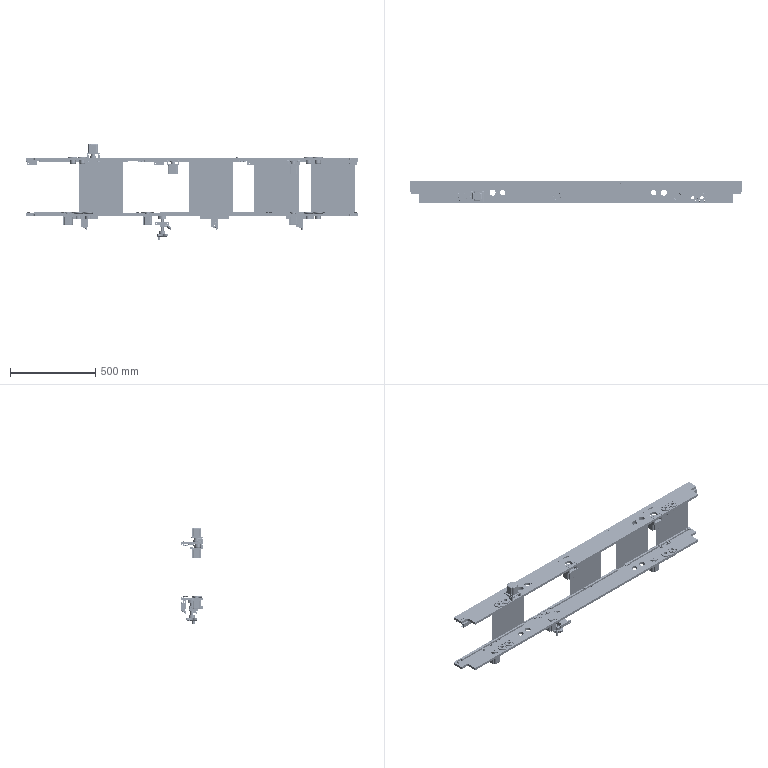Assembly | SolidWorks | mm | 127 component files | 127 solids | 6871 faces | box 1950 x 128 x 564.8 mm | volume 9759573 mm3 | cylinder 2934 | plane 2677 | torus 620 | cone 572 | spline 56 | sphere 12 | commonest cylinder face diameters 5 x216 7 x210 14 x194 63 x180 5.5 x170 4 x161 3.3 x158 10 x138
Bill of materials:
SL010-02047843SupportBar1-1 | 1 | White POM | Long, slender straight bar with a rectangular cross-section. It has three round holes through its wider face: one near each end and one at the middle.
SL010-02047843SupportBar1-1 | 3 | White POM | Long, slender straight bar of rectangular section with three through holes along its length: one near each end and one at the middle.
SL010-02047844SupportBar2-1 | 2 | White POM | Long, slender straight bar of rectangular section with three through holes, one near each end and one at the center. It looks essentially the same as unnamed part.
SL010-02047858StopBarNo.3-1 | 2 | White POM | Long rectangular bar with angled chamfers at both ends of one long edge. The middle section is reduced in height, giving a stepped recess. Four small elongated holes or slots pass through the wide side face.
SL010-02047858StopBarNo.4-1 | 1 | White POM | Long rectangular bar with angled end chamfers, four small elongated holes through the wide face, and a reduced-height recessed section offset toward one end.
SL010-B602-1 | 1 | 45 | Thick annular ring with a central through bore and a concentric annular groove cut into one flat face. The opposite face is flat.
SL010-_CLDM5_25_B_1_2-1 | 1 |  | Stepped cylindrical pin: a long small-diameter shank, a larger cylindrical collar, and a medium-diameter section ending in a hexagonal socket recess. The ends are chamfered or rounded.
SL010-_CLDM5_8_B_2_4-1 | 1 |  | Lever or crank arm: a cylindrical hub with a through bore, joined to a flat, tapered, curved arm that ends in a rounded tip.
SL010-HBA41-D63-1 | 1 |  | Wheel or knob with a finely toothed or knurled rim, a raised split-clamp hub with a central bore, and an off-center cylindrical pin on the underside.
SL010-LXFB-0102009-1 | 1 | Aluminum-6061 | Flanged ring or collar with a stepped (counterbored) central bore and four through holes equally spaced on a bolt circle. The outer edges are chamfered.
SL010-LXFB-0102010-1 | 1 | S45C | Rectangular plate block with a stepped, flanged (T-shaped) profile. The upper body has a large counterbored hole and two small holes. The wider base flange has horizontal through holes at its ends. The top corners are chamfered.
SL010-LXFB-0102011-1 | 1 | Aluminum-6061 | Rectangular block shaft clamp with a large through bore. A slit runs from the bore to one end, and a slot extends partway toward the other end. The block also has two through holes and a cross hole through the side, perpendicular to the slit.
SL010-LXFB-0102017-1 | 1 | S45C | Stepped cylindrical shaft: a long main section with reduced-diameter journals at both ends. One end has a circumferential groove near the tip.
SL010-C-LHFR20-2-1 | 8 |  | Flanged cylindrical bushing: a round flange with four through holes evenly spaced around a central through bore, and a plain cylindrical shank below it.
SL010-LXFB-010203-002-1 | 1 | Aluminum-6061 | Long, thin, flat plate with stepped or notched ends and a row of features along its length: several larger circular holes, many small holes and a few short slots.
SL010-LeadshineStepper-2-1 | 6 |  | Box-like body with a square front flange (chamfered corners) and a through hole at each corner, a raised circular boss in the middle, and a single cylindrical shaft sticking out of the boss.
SL010-LXFB-020200-007-1 | 3 | S45C | Pulley-like rotational part: a cylindrical body between two thin raised rims, a smaller cylindrical hub on one side with two radial holes in a line, and a small central through bore.
SL010-FL625ZZ-1 | 48 |  | Stepped annular part: a thin, wider base flange under a taller cylindrical ring with rounded top edge, a central through bore with a raised inner ring, and a shallow annular groove near the outer top edge.
SL010-LXFB-020200-020-1 | 3 | Aluminum-6061 | Flat T-shaped plate: a wide top bar with angled upper corners, and a narrower central stem with two holes in a line; inner corners are filleted. Edge views show a step in thickness or a joggle between the bar and the stem.
SL010-Material | 4 |  | Thin, plain rectangular sheet with no visible holes or features.
SL010-0ALk-010000-006-2-1 | 3 | 45 | Pulley-like rotational part: a cylindrical band between two thin rims, a smaller coaxial hub with two radial holes in a line, a chamfered hub end, and a small central through bore.
SL010-LXFB-0102007-1 | 3 | Aluminum-6061 | Square flat plate with small corner chamfers, a large central circular opening, four smaller through holes and four larger through holes.
SL010-LXFB-0102008-1 | 6 | Aluminum-6061 | Rectangular block with chamfered edges and two parallel through holes in its top face.
SL010-GB6171-86 M4-1 | 1 |  | Hexagonal nut-like part: chamfered on both faces, with a central round through bore.
SL010-LXFB-010202-003-1 | 2 | S45C | Long, slender bar with a rectangular cross-section, three small elongated holes through the narrow face (one at each end and one at mid-length), and angled cuts at the ends.
SL010-LXFB-010202-01 | 1 | S45C | Long, slender solid bar with a rectangular cross-section. It has three small slotted holes through one face, one near each end and one at mid-length. The bottom corners at both ends are chamfered or beveled.
SL010-LXFB-010203-01 | 1 | Aluminum-6061 | Long, thin flat plate with a rectangular notch or step at each end. Along the plate are three groups of round holes of different sizes, short slots, and many small holes. The pattern looks symmetric about the middle.
SL010-0ALk-010000-012-2-1 | 4 | 304 | Bracket bent from a uniform-thickness sheet into a C or U shape: a long top flange, a vertical web, and a shorter bottom flange. The top flange has a long slot with rounded ends. The web has a square cutout. The bottom flange has a single round hole, which may be countersunk or counterbored.
SL010-E3Z_D61-1 | 4 |  | Rectangular block body with a cylindrical stub on one end. A long, thin rod or cable extends from the body at an angle. There are two round through holes on the top face, and small cylindrical bosses and a rounded tab on one side face. The body outline has one chamfered corner.
Mates:
1. coincident | SL010-RightStreamline-1-1/SL010-LXFB-010203-01-1 face at (-975, -109.904, -316.035) dir (0, 1, 0) | SL010-LeftStreamline-1-1/SL010-LXFB-010203-002-1-1 face at (975, -109.904, -658.035) dir (0, 1, 0)
2. coincident | SL010-RightStreamline-1-1/SL010-LXFB-010203-01-1 face at (-975, -109.904, -316.035) dir (-1, 0, 0) | SL010-LeftStreamline-1-1/SL010-LXFB-010203-002-1-1 face at (-975, -109.904, -658.035) dir (-1, 0, 0)
3. distance | SL010-LeftStreamline-1-1/SL010-LXFB-010203-002-1-1 face at (0, -169.404, -643.035) dir (0, 0, 1) | SL010-RightStreamline-1-1/SL010-LXFB-010203-01-1 face at (0, -169.404, -331.035) dir (0, 0, -1)
4. coincident | SL010-Material-2 face at (110, -107.904, -487.035) dir (0, 1, 0) | SL010-Material-1 face at (-535, -107.904, -487.035) dir (0, 1, 0)
5. coincident | SL010-Material-2 face at (-12, -108.004, -345.035) dir (0, 0, -1) | SL010-Material-1 face at (-657, -108.004, -345.035) dir (0, 0, -1)
6. distance | SL010-RightStreamline-1-1/SL010-02047843SupportBar1-1-1 face at (898.47, -111.404, -341.035) dir (0, 1, 0) | SL010-Material-4 face at (827.087, -109.904, -487.035) dir (0, -1, 0)
7. width | SL010-Material-4 face at (697.087, -107.904, -637.035) dir (0, 0, -1) | SL010-Material-4 face at (697.087, -107.904, -337.035) dir (0, 0, 1) | SL010-RightStreamline-1-1/SL010-LXFB-010203-01-1 face at (0, -169.404, -316.035) dir (0, 0, 1) | SL010-LeftStreamline-1-1/SL010-LXFB-010203-002-1-1 face at (0, -169.404, -658.035) dir (0, 0, -1)
8. coincident | SL010-Material-4 face at (827.087, -107.904, -487.035) dir (0, 1, 0) | SL010-Material-2 face at (110, -107.904, -487.035) dir (0, 1, 0)
9. coincident | SL010-Material-4 edge at (705.087, -107.904, -345.035) dir (1, 0, 0) | SL010-Material-2 face at (-12, -108.004, -345.035) dir (0, 0, -1)
10. coincident | SL010-Material-4 face at (827.087, -107.904, -487.035) dir (0, 1, 0) | SL010-Material-3 face at (496.654, -107.904, -487.035) dir (0, 1, 0)
11. coincident | SL010-Material-4 face at (705.087, -108.004, -345.035) dir (0, 0, -1) | SL010-Material-3 edge at (374.654, -108.004, -345.035) dir (1, 0, 0)
12. concentric | SL010-LXFB-010203-002-1-1 face at (732.973, 100.193, 1492.5) dir (0, 0, -1) r 2.1 | SL010-PulleyAssembly-1-1/SL010-FL625ZZ-1-2 face at (732.973, 100.193, 1470.5) dir (0, 0, 1) r 2.5
13. distance | SL010-PulleyAssembly-1-1/SL010-FL625ZZ-1-1 face at (732.881, 107.193, 1491.5) dir (0, 0, 1) | SL010-LXFB-010203-002-1-1 face at (-227.027, 50.193, 1492.5) dir (0, 0, -1)
14. concentric | SL010-LXFB-010203-002-1-1 face at (532.973, 84.193, 1492.5) dir (0, 0, -1) r 2.1 | SL010-PulleyAssembly-1-2/SL010-FL625ZZ-1-2 face at (532.973, 84.193, 1470.5) dir (0, 0, 1) r 2.5
15. coincident | SL010-PulleyAssembly-1-1/SL010-FL625ZZ-1-2 face at (733.036, 107.193, 1481.5) dir (0, 0, -1) | SL010-PulleyAssembly-1-2/SL010-FL625ZZ-1-2 face at (533.02, 91.193, 1481.5) dir (0, 0, -1)
16. coincident | SL010-PulleyAssembly-1-1/SL010-FL625ZZ-1-2 face at (733.036, 107.193, 1481.5) dir (0, 0, -1) | SL010-PulleyAssembly-1-3/SL010-FL625ZZ-1-2 face at (473.371, 91.182, 1481.5) dir (0, 0, -1)
17. slot | SL010-PulleyAssembly-1-3/SL010-FL625ZZ-1-2 face at (472.973, 84.193, 1470.5) dir (0, 0, 1) r 2.5 | SL010-LXFB-010203-002-1-1 face at (455.723, 84.193, 1507.5) dir (0, 0, 1) r 2.75
18. coincident | SL010-PulleyAssembly-1-1/SL010-FL625ZZ-1-2 face at (733.036, 107.193, 1481.5) dir (0, 0, -1) | SL010-PulleyAssembly-1-7/SL010-FL625ZZ-1-2 face at (31.14, 94.439, 1481.5) dir (0, 0, -1)
19. slot | SL010-PulleyAssembly-1-13/SL010-FL625ZZ-1-2 face at (3.973, 84.193, 1470.5) dir (0, 0, 1) r 2.5 | SL010-LXFB-010203-002-1-1 face at (-13.277, 81.443, 1507.5) dir (0, 1, 0)
20. concentric | SL010-LXFB-010203-002-1-1 face at (-668.027, 100.193, 1492.5) dir (0, 0, -1) r 2.1 | SL010-PulleyAssembly-1-8/SL010-FL625ZZ-1-2 face at (-668.027, 100.193, 1470.5) dir (0, 0, 1) r 2.5
21. concentric | SL010-LXFB-010203-002-1-1 face at (-687.027, 100.193, 1492.5) dir (0, 0, -1) r 2.1 | SL010-PulleyAssembly-1-9/SL010-FL625ZZ-1-2 face at (-687.027, 100.193, 1470.5) dir (0, 0, 1) r 2.5
22. coincident | SL010-PulleyAssembly-1-1/SL010-FL625ZZ-1-2 face at (733.036, 107.193, 1481.5) dir (0, 0, -1) | SL010-PulleyAssembly-1-8/SL010-FL625ZZ-1-2 face at (-667.964, 107.193, 1481.5) dir (0, 0, -1)
23. coincident | SL010-PulleyAssembly-1-1/SL010-FL625ZZ-1-2 face at (733.036, 107.193, 1481.5) dir (0, 0, -1) | SL010-PulleyAssembly-1-6/SL010-FL625ZZ-1-2 face at (88.551, 106.566, 1481.5) dir (0, 0, -1)
24. concentric | SL010-LXFB-010203-002-1-1 face at (63.973, 84.193, 1492.5) dir (0, 0, -1) r 2.1 | SL010-PulleyAssembly-1-12/SL010-FL625ZZ-1-2 face at (63.973, 84.193, 1470.5) dir (0, 0, 1) r 2.5
25. coincident | SL010-PulleyAssembly-1-1/SL010-FL625ZZ-1-2 face at (733.036, 107.193, 1481.5) dir (0, 0, -1) | SL010-PulleyAssembly-1-12/SL010-FL625ZZ-1-2 face at (64.036, 91.193, 1481.5) dir (0, 0, -1)
26. coincident | SL010-PulleyAssembly-1-1/SL010-FL625ZZ-1-2 face at (733.036, 107.193, 1481.5) dir (0, 0, -1) | SL010-PulleyAssembly-1-13/SL010-FL625ZZ-1-2 face at (4.977, 91.121, 1481.5) dir (0, 0, -1)
27. coincident | SL010-PulleyAssembly-1-1/SL010-FL625ZZ-1-2 face at (733.036, 107.193, 1481.5) dir (0, 0, -1) | SL010-PulleyAssembly-1-9/SL010-FL625ZZ-1-2 face at (-693.737, 98.198, 1481.5) dir (0, 0, -1)
28. concentric | SL010-LXFB-010203-002-1-1 face at (-942.027, 84.193, 1492.5) dir (0, 0, -1) r 2.1 | SL010-PulleyAssembly-1-14/SL010-FL625ZZ-1-2 face at (-942.027, 84.193, 1470.5) dir (0, 0, 1) r 2.5
29. coincident | SL010-PulleyAssembly-1-1/SL010-FL625ZZ-1-2 face at (733.036, 107.193, 1481.5) dir (0, 0, -1) | SL010-PulleyAssembly-1-14/SL010-FL625ZZ-1-2 face at (-943.982, 90.915, 1481.5) dir (0, 0, -1)
30. slot | SL010-PulleyAssembly-1-15/SL010-FL625ZZ-1-1 face at (-1002.027, 84.193, 1502.5) dir (0, 0, -1) r 2.5 | SL010-LXFB-010203-002-1-1 face at (-1019.277, 84.193, 1507.5) dir (0, 0, 1) r 2.75
31. coincident | SL010-PulleyAssembly-1-1/SL010-FL625ZZ-1-2 face at (733.036, 107.193, 1481.5) dir (0, 0, -1) | SL010-PulleyAssembly-1-15/SL010-FL625ZZ-1-2 face at (-1006.227, 89.793, 1481.5) dir (0, 0, -1)
32. concentric | SL010-LXFB-010203-002-1-1 face at (-1187.027, 100.193, 1492.5) dir (0, 0, -1) r 2.1 | SL010-PulleyAssembly-1-18/SL010-FL625ZZ-1-2 face at (-1187.027, 100.193, 1470.5) dir (0, 0, 1) r 2.5
33. coincident | SL010-PulleyAssembly-1-1/SL010-FL625ZZ-1-2 face at (733.036, 107.193, 1481.5) dir (0, 0, -1) | SL010-PulleyAssembly-1-18/SL010-FL625ZZ-1-2 face at (-1186.964, 107.193, 1481.5) dir (0, 0, -1)
34. coincident | SL010-LXFB-010203-002-1-1 face at (-227.027, 50.193, 1492.5) dir (0, 0, -1) | SL010-02047844SupportBar2-1-1 face at (-316.451, 103.193, 1492.5) dir (0, 0, 1)
35. distance | SL010-02047844SupportBar2-1-1 face at (-36.451, 108.193, 1482.5) dir (0, 1, 0) | SL010-LXFB-010203-002-1-1 face at (-1202.027, 109.693, 1507.5) dir (0, 1, 0)
36. symmetric | SL010-PulleyAssembly-1-7/SL010-FL625ZZ-1-1 face at (35.126, 100.193, 1502.5) dir (0, 0, -1) r 8 | SL010-PulleyAssembly-1-8/SL010-FL625ZZ-1-1 face at (-668.027, 100.193, 1502.5) dir (0, 0, -1) r 8 | SL010-02047844SupportBar2-1-1 plane at (-316.451, 103.193, 1487.5) dir (-1, 0, 0)
37. coincident | SL010-02047843SupportBar1-1-1 face at (-937.027, 103.193, 1482.5) dir (0, 0, -1) | SL010-02047844SupportBar2-1-1 face at (-316.451, 103.193, 1482.5) dir (0, 0, -1)
38. coincident | SL010-02047843SupportBar1-1-1 face at (-697.027, 108.193, 1482.5) dir (0, 1, 0) | SL010-02047844SupportBar2-1-1 face at (-36.451, 108.193, 1482.5) dir (0, 1, 0)
39. symmetric | SL010-PulleyAssembly-1-9/SL010-FL625ZZ-1-1 face at (-687.027, 100.193, 1502.5) dir (0, 0, -1) r 8 | SL010-PulleyAssembly-1-18/SL010-FL625ZZ-1-1 face at (-1187.027, 100.193, 1502.5) dir (0, 0, -1) r 8 | SL010-02047843SupportBar1-1-1 plane at (-937.027, 103.193, 1487.5) dir (-1, 0, 0)
40. concentric | SL010-LXFB-010203-002-1-1 face at (-64.755, 67.421, 1507.5) dir (0, 0, 1) r 2.1 | SL010-2M-0112-000-2-1-1/SL010-LXFB-0102009-1-1 face at (-64.755, 67.421, 1522.5) dir (0, 0, 1) r 2.75
41. concentric | SL010-LXFB-010203-002-1-1 face at (-39.299, 67.421, 1507.5) dir (0, 0, 1) r 2.1 | SL010-2M-0112-000-2-1-1/SL010-LXFB-0102009-1-1 face at (-39.299, 67.421, 1522.5) dir (0, 0, 1) r 5
42. coincident | SL010-LXFB-010203-002-1-1 face at (-227.027, 50.193, 1507.5) dir (0, 0, 1) | SL010-2M-0112-000-2-1-1/SL010-LXFB-0102009-1-1 face at (-52.027, 54.693, 1507.5) dir (0, 0, -1)
43. coincident | SL010-LXFB-010203-002-1-1 face at (-227.027, 50.193, 1507.5) dir (0, 0, 1) | SL010-MotorDriveWheel-1-1/SL010-LeadshineStepper-2-1-1 face at (531.173, -0.05689, 1507.5) dir (0, 0, -1)
44. distance | SL010-MotorDriveWheel-1-1/SL010-LeadshineStepper-2-1-1 face at (474.773, 56.343, 1561.5) dir (0, 1, 0) | SL010-LXFB-010203-002-1-1 face at (-1202.027, 109.693, 1507.5) dir (0, 1, 0)
45. coincident | SL010-LXFB-010203-002-1-1 face at (-227.027, 50.193, 1507.5) dir (0, 0, 1) | SL010-MotorDriveWheel-1-2/SL010-LeadshineStepper-2-1-1 face at (62.173, -0.05689, 1507.5) dir (0, 0, -1)
46. coincident | SL010-MotorDriveWheel-1-1/SL010-LeadshineStepper-2-1-1 face at (474.773, 56.343, 1561.5) dir (0, 1, 0) | SL010-MotorDriveWheel-1-2/SL010-LeadshineStepper-2-1-1 face at (5.773, 56.343, 1561.5) dir (0, 1, 0)
47. coincident | SL010-LXFB-010203-002-1-1 face at (-227.027, 50.193, 1507.5) dir (0, 0, 1) | SL010-MotorDriveWheel-1-3/SL010-LeadshineStepper-2-1-1 face at (-793.827, -0.05689, 1507.5) dir (0, 0, -1)
48. coincident | SL010-LXFB-010203-002-1-1 face at (-227.027, 50.193, 1492.5) dir (0, 0, -1) | SL010-02047843SupportBar1-1-2 face at (442.147, 103.193, 1492.5) dir (0, 0, 1)
49. coincident | SL010-02047844SupportBar2-1-1 face at (-36.451, 108.193, 1482.5) dir (0, 1, 0) | SL010-02047843SupportBar1-1-2 face at (702.147, 108.193, 1482.5) dir (0, 1, 0)
50. coincident | SL010-LXFB-010203-002-1-1 face at (-227.027, 50.193, 1507.5) dir (0, 0, 1) | SL010-02047858StopBarNo.3-1-1 face at (747.973, 109.693, 1507.5) dir (0, 0, 1)
51. coincident | SL010-LXFB-010203-002-1-1 face at (-1202.027, 109.693, 1507.5) dir (0, 1, 0) | SL010-02047858StopBarNo.3-1-1 face at (406.473, 109.693, 1497) dir (0, -1, 0)
52. coincident | SL010-LXFB-010203-002-1-1 face at (747.973, 109.693, 1507.5) dir (1, 0, 0) | SL010-02047858StopBarNo.3-1-1 face at (747.973, 109.693, 1486.5) dir (1, 0, 0)
53. coincident | SL010-LXFB-010203-002-1-1 face at (-227.027, 50.193, 1507.5) dir (0, 0, 1) | SL010-02047858StopBarNo.3-1-2 face at (-519.027, 109.693, 1507.5) dir (0, 0, 1)
54. coincident | SL010-LXFB-010203-002-1-1 face at (-1202.027, 109.693, 1507.5) dir (0, 1, 0) | SL010-02047858StopBarNo.3-1-2 face at (-860.527, 109.693, 1497) dir (0, -1, 0)
55. coincident | SL010-LXFB-010203-002-1-1 face at (-1202.027, 109.693, 1507.5) dir (-1, 0, 0) | SL010-02047858StopBarNo.3-1-2 face at (-1202.027, 109.693, 1486.5) dir (-1, 0, 0)
56. coincident | SL010-02047858StopBarNo.3-1-1 face at (406.473, 117.693, 1497) dir (0, 1, 0) | SL010-02047858StopBarNo.4-1-2 face at (-227.027, 117.693, 1497) dir (0, 1, 0)
57. coincident | SL010-02047858StopBarNo.3-1-1 face at (64.973, 109.693, 1486.5) dir (-1, 0, 0) | SL010-02047858StopBarNo.4-1-2 face at (64.973, 117.693, 1486.5) dir (1, 0, 0)
58. coincident | SL010-LXFB-010203-002-1-1 face at (-227.027, 50.193, 1507.5) dir (0, 0, 1) | SL010-02047858StopBarNo.4-1-2 face at (-519.027, 117.693, 1507.5) dir (0, 0, 1)
59. coincident | SL010-LXFB-010203-002-1-1 face at (-227.027, 50.193, 1507.5) dir (0, 0, 1) | SL010-SideClampAssembly-DB-1-1/SL010-HLQ8X10SAF(0)+(DS1-H-2)-DB-1-1/SL010-HLQ8X10-S-AF-0-rod-DB-1-1 face at (414.973, 103.693, 1507.5) dir (0, 0, -1)
60. distance | SL010-SideClampAssembly-DB-1-1/SL010-LXFB-020200-020-1-1 face at (406.473, 110.193, 1531.5) dir (0, -1, 0) | SL010-LXFB-010203-002-1-1 face at (-1202.027, 109.693, 1507.5) dir (0, 1, 0)
61. width | SL010-SideClampAssembly-DB-1-1/SL010-LXFB-020200-020-1-1 face at (322.723, 116.193, 1570.5) dir (-1, 0, 0) | SL010-SideClampAssembly-DB-1-1/SL010-LXFB-020200-020-1-1 face at (490.223, 116.193, 1570.5) dir (1, 0, 0) | SL010-02047858StopBarNo.3-1-1 face at (321.723, 109.693, 1507.5) dir (1, 0, 0) | SL010-02047858StopBarNo.3-1-1 face at (491.223, 109.693, 1507.5) dir (-1, 0, 0)
62. coincident | SL010-SideClampAssembly-DB-1-1/SL010-LXFB-020200-020-1-1 face at (406.473, 116.193, 1531.5) dir (0, 1, 0) | SL010-SideClampAssembly-DB-1-2/SL010-LXFB-020200-020-1-1 face at (-358.277, 116.193, 1531.5) dir (0, 1, 0)
63. coincident | SL010-LXFB-010203-002-1-1 face at (-227.027, 50.193, 1507.5) dir (0, 0, 1) | SL010-SideClampAssembly-DB-1-2/SL010-HLQ8X10SAF(0)+(DS1-H-2)-DB-1-1/SL010-HLQ8X10-S-AF-0-rod-DB-1-1 face at (-349.777, 103.693, 1507.5) dir (0, 0, -1)
64. width | SL010-SideClampAssembly-DB-1-2/SL010-LXFB-020200-020-1-1 face at (-442.027, 116.193, 1570.5) dir (-1, 0, 0) | SL010-SideClampAssembly-DB-1-2/SL010-LXFB-020200-020-1-1 face at (-274.527, 116.193, 1570.5) dir (1, 0, 0) | SL010-02047858StopBarNo.4-1-2 face at (-273.527, 110.554, 1486.5) dir (-1, 0, 0) | SL010-02047858StopBarNo.4-1-2 face at (-443.027, 110.554, 1486.5) dir (1, 0, 0)
65. coincident | SL010-SideClampAssembly-DB-1-2/SL010-LXFB-020200-020-1-1 face at (-358.277, 116.193, 1531.5) dir (0, 1, 0) | SL010-SideClampAssembly-DB-1-3/SL010-LXFB-020200-020-1-1 face at (-860.527, 116.193, 1531.5) dir (0, 1, 0)
66. coincident | SL010-LXFB-010203-002-1-1 face at (-227.027, 50.193, 1507.5) dir (0, 0, 1) | SL010-SideClampAssembly-DB-1-3/SL010-HLQ8X10SAF(0)+(DS1-H-2)-DB-1-1/SL010-HLQ8X10-S-AF-0-rod-DB-1-1 face at (-852.027, 103.693, 1507.5) dir (0, 0, -1)
67. width | SL010-SideClampAssembly-DB-1-3/SL010-LXFB-020200-020-1-1 face at (-944.277, 116.193, 1570.5) dir (-1, 0, 0) | SL010-SideClampAssembly-DB-1-3/SL010-LXFB-020200-020-1-1 face at (-776.777, 116.193, 1570.5) dir (1, 0, 0) | SL010-02047858StopBarNo.3-1-2 face at (-945.277, 109.693, 1507.5) dir (1, 0, 0) | SL010-02047858StopBarNo.3-1-2 face at (-775.777, 109.693, 1507.5) dir (-1, 0, 0)
68. concentric | SL010-LXFB-010203-002-1-1 face at (-912.027, 19.693, 1492.5) dir (0, 0, 1) r 16 | SL010-C-LHFR20-2-1-1 face at (-912.027, 19.693, 1526.5) dir (0, 0, -1) r 16
69. concentric | SL010-LXFB-010203-002-1-1 face at (-896.825, 34.896, 1507.5) dir (0, 0, 1) r 2.1 | SL010-C-LHFR20-2-1-1 face at (-896.825, 34.896, 1484.5) dir (0, 0, -1) r 4.5
70. coincident | SL010-LXFB-010203-002-1-1 face at (-227.027, 50.193, 1492.5) dir (0, 0, -1) | SL010-C-LHFR20-2-1-1 edge at (-912.027, 19.693, 1492.5) dir (0, 0, -1) r 26.5
71. concentric | SL010-LXFB-010203-002-1-1 face at (-967.027, 19.693, 1492.5) dir (0, 0, 1) r 16 | SL010-C-LHFR20-2-1-2 face at (-967.027, 19.693, 1526.5) dir (0, 0, -1) r 16
72. concentric | SL010-LXFB-010203-002-1-1 face at (-951.825, 34.896, 1507.5) dir (0, 0, 1) r 2.1 | SL010-C-LHFR20-2-1-2 face at (-951.825, 34.896, 1484.5) dir (0, 0, -1) r 4.5
73. coincident | SL010-LXFB-010203-002-1-1 face at (-227.027, 50.193, 1492.5) dir (0, 0, -1) | SL010-C-LHFR20-2-1-2 face at (-955.89, 30.83, 1492.5) dir (0, 0, 1)
74. coincident | SL010-LXFB-010203-002-1-1 face at (-227.027, 50.193, 1492.5) dir (0, 0, -1) | SL010-C-LHFR20-2-1-4 face at (334.11, 30.83, 1492.5) dir (0, 0, 1)
75. coincident | SL010-LXFB-010203-002-1-1 face at (-227.027, 50.193, 1492.5) dir (0, 0, -1) | SL010-C-LHFR20-2-1-3 face at (279.11, 30.83, 1492.5) dir (0, 0, 1)
76. concentric | SL010-LXFB-010203-002-1-1 sketch segment at (3.973, 84.193, 1492.5) dir (0, 0, -1) r 9.639 | SL010-PulleyAssembly-1-13/SL010-FL625ZZ-1-2 face at (3.973, 84.193, 1470.5) dir (0, 0, 1) r 2.5
77. concentric | SL010-LXFB-010203-002-1-1 sketch segment at (-1002.027, 84.193, 1492.5) dir (0, 0, -1) r 11.985 | SL010-PulleyAssembly-1-15/SL010-FL625ZZ-1-2 face at (-1002.027, 84.193, 1470.5) dir (0, 0, 1) r 2.5
78. concentric | SL010-LXFB-010203-002-1-1 sketch segment at (472.973, 84.193, 1492.5) dir (0, 0, -1) r 10.481 | SL010-PulleyAssembly-1-3/SL010-FL625ZZ-1-2 face at (472.973, 84.193, 1470.5) dir (0, 0, 1) r 2.5
79. symmetric | SL010-PulleyAssembly-1-12/SL010-FL625ZZ-1-1 face at (63.973, 84.193, 1502.5) dir (0, 0, -1) r 8 | SL010-PulleyAssembly-1-13/SL010-FL625ZZ-1-1 face at (3.973, 84.193, 1502.5) dir (0, 0, -1) r 8 | SL010-MotorDriveWheel-1-2/SL010-LeadshineStepper-2-1-1 plane at (33.973, 28.143, 1507.5) dir (-1, 0, 0)
80. symmetric | SL010-PulleyAssembly-1-2/SL010-FL625ZZ-1-1 face at (532.973, 84.193, 1502.5) dir (0, 0, -1) r 8 | SL010-PulleyAssembly-1-3/SL010-FL625ZZ-1-1 face at (472.973, 84.193, 1502.5) dir (0, 0, -1) r 8 | SL010-MotorDriveWheel-1-1/SL010-LeadshineStepper-2-1-1 plane at (502.973, 28.143, 1507.5) dir (-1, 0, 0)
81. concentric | SL010-LXFB-010203-002-1-1 face at (-822.027, 28.143, 1507.5) dir (0, 0, -1) r 22.5 | SL010-MotorDriveWheel-1-3/SL010-LXFB-020200-007-1-1 face at (-822.027, 28.143, 1491.9) dir (0, 0, 1) r 18.5
82. coincident | SL010-LXFB-0102009-1-1 face at (0, 25, 37) dir (0, 0, 1) | SL010-B602-1-1 face at (0, 38.7, 37) dir (0, 0, -1)
83. concentric | SL010-LXFB-0102009-1-1 face at (0, 25, 37) dir (0, 0, 1) r 14 | SL010-B602-1-1 face at (0, 25, 45) dir (0, 0, -1) r 6
84. concentric | SL010-B602-1-1 face at (0, 25, 45) dir (0, 0, -1) r 6 | SL010-LXFB-0102017-1-2 face at (0, 25, 37) dir (0, 0, 1) r 6
85. coincident | SL010-B602-1-1 face at (0, 33.8, 37) dir (0, 0, -1) | SL010-LXFB-0102017-1-2 face at (0, 25, 37) dir (0, 0, 1)
86. concentric | SL010-LXFB-0102017-1-2 face at (0, 25, -43) dir (0, 0, 1) r 8 | SL010-LXFB-0102010-1-1 face at (0, 25, 10) dir (0, 0, 1) r 8
87. distance | SL010-LXFB-0102010-1-1 face at (0, 0, -10) dir (0, 0, -1) | SL010-LXFB-0102009-1-1 face at (0, 25, 30) dir (0, 0, -1)
88. coincident | SL010-LXFB-0102010-1-1 face at (0, 0, -10) dir (0, 0, -1) | SL010-LXFB-0102011-1-1 face at (0, 16.5, -10) dir (0, 0, 1)
89. concentric | SL010-LXFB-0102017-1-2 face at (0, 25, -43) dir (0, 0, 1) r 8 | SL010-LXFB-0102011-1-1 face at (0, 25, -20) dir (0, 0, 1) r 8
90. parallel | SL010-LXFB-0102010-1-1 face at (-25, 40, 10) dir (0, 1, 0) | SL010-LXFB-0102011-1-1 face at (-15, 41.5, -10) dir (0, 1, 0)
91. coordinate | SL010-LXFB-0102010-1-1 sketch point at (0, 0, 0) dir (1, 0, 0) | SL010-2M-0112-000-2-1 sketch point at (0, 0, 0) dir (1, 0, 0)
92. angle | SL010-LXFB-0102009-1-1 plane at (0, 25, 30) dir (-0.7071, 0.7071, 0) | SL010-LXFB-0102010-1-1 face at (-25, 40, 10) dir (0, 1, 0)
93. concentric | SL010-LXFB-0102011-1-1 face at (-1.5, 36.5, -15) dir (1, 0, 0) r 2.5 | SL010-CLDM5_25_B-1-1/SL010-_CLDM5_25_B_1_2-1-1 face at (-10, 36.5, -15) dir (1, 0, 0) r 2.5
94. coincident | SL010-LXFB-0102011-1-1 face at (15, 41.5, -10) dir (1, 0, 0) | SL010-CLDM5_25_B-1-1/SL010-_CLDM5_25_B_1_2-1-1 face at (15, 31.753, -16.572) dir (-1, 0, 0)
95. concentric | SL010-LXFB-0102017-1-2 face at (0, 25, -63) dir (0, 0, 1) r 6 | SL010-HBA41-D63-1-1 face at (0, 25, -43) dir (0, 0, -1) r 6
96. coincident | SL010-LXFB-0102017-1-2 face at (-5.653, 19.339, -43) dir (0, 0, -1) | SL010-HBA41-D63-1-1 face at (2.778, 19.682, -43) dir (0, 0, 1)
97. distance | SL010-LXFB-020200-007-1-1 face at (-19.454, -2.727, 74.6) dir (1, 0, 0) | SL010-LeadshineStepper-2-1-1 face at (-18.454, -2.727, 74.6) dir (-1, 0, 0)
98. concentric | SL010-FL625ZZ-1-1 face at (-20.536, 14.936, 0) dir (-1, 0, 0) r 2.5 | SL010-FL625ZZ-1-2 face at (-52.536, 14.936, 0) dir (1, 0, 0) r 2.5
99. coincident | SL010-FL625ZZ-1-1 face at (-36.536, 22.636, 0) dir (-1, 0, 0) | SL010-FL625ZZ-1-2 face at (-36.536, 22.634, -0.1708) dir (1, 0, 0)
100. coincident | SL010-LXFB-020200-020-1-1 face at (53, -25.015, 30) dir (0, 0, -1) | SL010-HLQ8X10SAF(0)+(DS1-H-2)-DB-1-1/SL010-HLQ8X10-S-AF-0-H-2-body-DB-1-1 face at (14, -45.015, 30) dir (0, 0, 1)
101. width | SL010-HLQ8X10SAF(0)+(DS1-H-2)-DB-1-1/SL010-HLQ8X10-S-AF-0-H-2-body-DB-1-1 face at (14, -5.015, 30) dir (0, 1, 0) | SL010-HLQ8X10SAF(0)+(DS1-H-2)-DB-1-1/SL010-HLQ8X10-S-AF-0-H-2-body-DB-1-1 face at (14, -45.015, 28) dir (0, -1, 0) | SL010-LXFB-020200-020-1-1 face at (60, -45.015, 30) dir (0, -1, 0) | SL010-LXFB-020200-020-1-1 face at (60, -5.015, 30) dir (0, 1, 0)
102. concentric | SL010-LXFB-020200-020-1-1 face at (21, -25.015, 36) dir (0, 0, 1) r 2.25 | SL010-HLQ8X10SAF(0)+(DS1-H-2)-DB-1-1/SL010-HLQ8X10-S-AF-0-H-2-body-DB-1-1 face at (21, -25.015, 30) dir (0, 0, -1) r 1.621
103. distance | SL010-HLQ8X10-S-AF-0-H-2-body-DB-1-1 plane at (0, 0, 0) dir (-1, 0, 0) | SL010-HLQ8X10-S-AF(0-H-2)-dummy-DB-1-1 plane at (0, 0, 0) dir (1, 0, 0)
104. coincident | SL010-HLQ8X10-S-AF(0-H-2)-dummy-DB-1-1 axis at (80.9, 0, 0) dir (-1, 0, 0) | SL010-HLQ8X10-S-AF-0-H-2-body-DB-1-1 axis at (-80.9, 0, 0) dir (1, 0, 0)
105. angle | SL010-HLQ8X10-S-AF-0-H-2-body-DB-1-1 plane at (0, 0, 0) dir (0, 0, -1) | SL010-HLQ8X10-S-AF(0-H-2)-dummy-DB-1-1 plane at (0, 0, 0) dir (0, 0, -1)
106. coincident | SL010-HLQ8X10-S-AF-0-H-2-body-DB-1-1 axis at (-80.9, 0, 0) dir (1, 0, 0) | SL010-HLQ8X10-S-AF-0-rod-DB-1-1 axis at (70.9, 0, 0) dir (-1, 0, 0)
107. angle | SL010-HLQ8X10-S-AF-0-rod-DB-1-1 plane at (-10, 0, 0) dir (0, 0, -1) | SL010-HLQ8X10-S-AF-0-H-2-body-DB-1-1 plane at (0, 0, 0) dir (0, 0, -1)
108. distance | SL010-DS1-H-DB-1-1 plane at (0, -16.65, -3) dir (-1, 0, 0) | SL010-HLQ8X10-S-AF-0-H-2-body-DB-1-1 plane at (0, 0, 0) dir (1, 0, 0)
109. coincident | SL010-HLQ8X10-S-AF-0-H-2-body-DB-1-1 axis at (80.9, -16.65, -3) dir (-1, 0, 0) | SL010-DS1-H-DB-1-1 axis at (-63.9, -16.65, -3) dir (1, 0, 0)
110. angle | SL010-DS1-H-DB-1-1 plane at (17, -16.65, -3) dir (0, 0, -1) | SL010-HLQ8X10-S-AF-0-H-2-body-DB-1-1 plane at (0, 0, -3) dir (0, 0, -1)
111. distance | SL010-DS1-H-DB-1-2 plane at (45.5, -16.65, 3.2) dir (1, 0, 0) | SL010-HLQ8X10-S-AF-0-H-2-body-DB-1-1 plane at (45.5, 0, 0) dir (1, 0, 0)
112. coincident | SL010-HLQ8X10-S-AF-0-H-2-body-DB-1-1 axis at (80.9, -16.65, 3.2) dir (-1, 0, 0) | SL010-DS1-H-DB-1-2 axis at (109.4, -16.65, 3.2) dir (-1, 0, 0)
113. angle | SL010-DS1-H-DB-1-2 plane at (28.5, -16.65, 3.2) dir (0, 0, 1) | SL010-HLQ8X10-S-AF-0-H-2-body-DB-1-1 plane at (0, 0, 3.2) dir (0, 0, -1)
114. distance | SL010-HLQ8X10-S-AF-0-H-2-body-DB-1-1 face at (0, -16.65, 3.2) dir (-1, 0, 0) | SL010-HLQ8X10-S-AF-0-rod-DB-1-1 face at (-11.5, -8.5, 0) dir (1, 0, 0)
115. coincident | SL010-PulleyAssembly-1-5/SL010-FL625ZZ-1-2 face at (295.762, 44.869, -329.5) dir (0, 0, 1) | SL010-PulleyAssembly-1-7/SL010-FL625ZZ-1-2 face at (630.044, 38.853, -329.5) dir (0, 0, 1)
116. coincident | SL010-PulleyAssembly-1-5/SL010-FL625ZZ-1-2 face at (295.762, 44.869, -329.5) dir (0, 0, 1) | SL010-PulleyAssembly-1-8/SL010-FL625ZZ-1-2 face at (565.821, 40.952, -329.5) dir (0, 0, 1)
117. coincident | SL010-PulleyAssembly-1-10/SL010-FL625ZZ-1-2 face at (305.499, 55.361, -329.5) dir (0, 0, 1) | SL010-PulleyAssembly-1-11/SL010-FL625ZZ-1-2 face at (-84.256, 27.803, -329.5) dir (0, 0, 1)
118. coincident | SL010-PulleyAssembly-1-11/SL010-FL625ZZ-1-2 face at (-84.256, 27.803, -329.5) dir (0, 0, 1) | SL010-PulleyAssembly-1-12/SL010-FL625ZZ-1-2 face at (-135.376, 38.168, -329.5) dir (0, 0, 1)
119. distance | SL010-PulleyAssembly-1-9/SL010-FL625ZZ-1-2 face at (-970.248, 46.013, -329.5) dir (0, 0, 1) | SL010-LXFB-010203-01-1 face at (0, 0, -328.5) dir (0, 0, -1)
120. coincident | SL010-PulleyAssembly-1-9/SL010-FL625ZZ-1-1 face at (-970.335, 46.142, -339.5) dir (0, 0, -1) | SL010-PulleyAssembly-1-13/SL010-FL625ZZ-1-1 face at (-603.337, 36.145, -339.5) dir (0, 0, -1)
121. concentric | SL010-LXFB-010203-01-1 face at (-610, 34, -313.5) dir (0, 0, 1) r 2.1 | SL010-PulleyAssembly-1-13/SL010-FL625ZZ-1-1 face at (-610, 34, -350.5) dir (0, 0, 1) r 2.5
122. slot | SL010-PulleyAssembly-1-14/SL010-FL625ZZ-1-1 face at (-550, 34, -350.5) dir (0, 0, 1) r 2.5 | SL010-LXFB-010203-01-1 face at (-532.75, 34, -313.5) dir (0, 0, 1) r 2.75
123. coincident | SL010-PulleyAssembly-1-9/SL010-FL625ZZ-1-1 face at (-970.335, 46.142, -339.5) dir (0, 0, -1) | SL010-PulleyAssembly-1-14/SL010-FL625ZZ-1-1 face at (-543.153, 35.457, -339.5) dir (0, 0, -1)
124. coincident | SL010-PulleyAssembly-1-17/SL010-FL625ZZ-1-1 face at (-303.337, 52.145, -339.5) dir (0, 0, -1) | SL010-PulleyAssembly-1-18/SL010-FL625ZZ-1-1 face at (-284.337, 52.145, -339.5) dir (0, 0, -1)
125. coincident | SL010-PulleyAssembly-1-9/SL010-FL625ZZ-1-1 face at (-970.335, 46.142, -339.5) dir (0, 0, -1) | SL010-PulleyAssembly-1-17/SL010-FL625ZZ-1-1 face at (-303.337, 52.145, -339.5) dir (0, 0, -1)
126. concentric | SL010-LXFB-010203-01-1 face at (-310, 50, -313.5) dir (0, 0, 1) r 2.1 | SL010-PulleyAssembly-1-17/SL010-FL625ZZ-1-1 face at (-310, 50, -350.5) dir (0, 0, 1) r 2.5
127. concentric | SL010-LXFB-010203-01-1 face at (-291, 50, -313.5) dir (0, 0, 1) r 2.1 | SL010-PulleyAssembly-1-18/SL010-FL625ZZ-1-1 face at (-291, 50, -350.5) dir (0, 0, 1) r 2.5
128. concentric | SL010-LXFB-010203-01-1 face at (-141, 34, -313.5) dir (0, 0, 1) r 2.1 | SL010-PulleyAssembly-1-12/SL010-FL625ZZ-1-2 face at (-141, 34, -318.5) dir (0, 0, -1) r 2.5
129. coincident | SL010-PulleyAssembly-1-9/SL010-FL625ZZ-1-1 face at (-970.335, 46.142, -339.5) dir (0, 0, -1) | SL010-PulleyAssembly-1-12/SL010-FL625ZZ-1-1 face at (-135.285, 38.042, -339.5) dir (0, 0, -1)
130. coincident | SL010-PulleyAssembly-1-11/SL010-FL625ZZ-1-1 face at (-84.392, 27.877, -339.5) dir (0, 0, -1) | SL010-PulleyAssembly-1-12/SL010-FL625ZZ-1-1 face at (-135.285, 38.042, -339.5) dir (0, 0, -1)
131. slot | SL010-PulleyAssembly-1-11/SL010-FL625ZZ-1-1 face at (-81, 34, -350.5) dir (0, 0, 1) r 2.5 | SL010-LXFB-010203-01-1 face at (-98.25, 31.25, -313.5) dir (0, 1, 0)
132. coincident | SL010-PulleyAssembly-1-5/SL010-FL625ZZ-1-1 face at (295.647, 44.765, -339.5) dir (0, 0, -1) | SL010-PulleyAssembly-1-11/SL010-FL625ZZ-1-1 face at (-84.392, 27.877, -339.5) dir (0, 0, -1)
133. concentric | SL010-LXFB-010203-01-1 face at (291, 50, -313.5) dir (0, 0, 1) r 2.1 | SL010-PulleyAssembly-1-5/SL010-FL625ZZ-1-1 face at (291, 50, -350.5) dir (0, 0, 1) r 2.5
134. distance | SL010-PulleyAssembly-1-1/SL010-FL625ZZ-1-2 face at (966.271, 42.522, -329.5) dir (0, 0, 1) | SL010-LXFB-010203-01-1 face at (0, 0, -328.5) dir (0, 0, -1)
135. slot | SL010-PulleyAssembly-1-7/SL010-FL625ZZ-1-1 face at (625, 34, -350.5) dir (0, 0, 1) r 2.5 | SL010-LXFB-010203-01-1 face at (607.75, 31.25, -313.5) dir (0, 1, 0)
136. concentric | SL010-LXFB-010203-01-1 face at (565, 34, -313.5) dir (0, 0, 1) r 2.1 | SL010-PulleyAssembly-1-8/SL010-FL625ZZ-1-1 face at (565, 34, -350.5) dir (0, 0, 1) r 2.5
137. concentric | SL010-LXFB-010203-01-1 face at (565, 34, -313.5) dir (0, 0, 1) r 2.1 | SL010-PulleyAssembly-1-8/SL010-FL625ZZ-1-2 face at (565, 34, -318.5) dir (0, 0, -1) r 2.5
138. distance | SL010-LXFB-010203-01-1 face at (-975, -59.5, -313.5) dir (0, -1, 0) | SL010-BeltMotorAssembly-1-1/SL010-LXFB-0102008-1-1 face at (-617.5, -58.5, -293.5) dir (0, -1, 0)
139. coincident | SL010-LXFB-010203-01-1 face at (0, 0, -328.5) dir (0, 0, -1) | SL010-BeltMotorAssembly-1-2/SL010-LXFB-0102008-1-1 face at (-78.5, -46, -328.5) dir (0, 0, 1)
140. distance | SL010-LXFB-010203-01-1 face at (-975, -59.5, -313.5) dir (0, -1, 0) | SL010-BeltMotorAssembly-1-2/SL010-LXFB-0102008-1-1 face at (-73.5, -58.5, -348.5) dir (0, -1, 0)
141. coincident | SL010-BeltMotorAssembly-1-2/SL010-LeadshineStepper-2-1-1 face at (-82.8, -50.25, -410.5) dir (0, 0, -1) | SL010-BeltMotorAssembly-1-3/SL010-LeadshineStepper-2-1-1 face at (623.2, -50.25, -410.5) dir (0, 0, -1)
142. distance | SL010-LXFB-010203-01-1 face at (-975, -59.5, -313.5) dir (0, -1, 0) | SL010-BeltMotorAssembly-1-3/SL010-LXFB-0102008-1-1 face at (632.5, -58.5, -348.5) dir (0, -1, 0)
143. coincident | SL010-LXFB-010203-01-1 face at (0, 0, -328.5) dir (0, 0, -1) | SL010-SensorAssembly-F-1-1/SL010-0ALk-010000-012-2-1-1 face at (940, 9, -328.5) dir (0, 0, 1)
144. slot | SL010-SensorAssembly-F-1-1/SL010-0ALk-010000-012-2-1-1 face at (920, 17, -329.7) dir (0, 1, 0) | SL010-LXFB-010203-01-1 face at (960, 19.5, -313.5) dir (0, 0, 1) r 1.25
145. slot | SL010-LXFB-010203-01-1 face at (945, 19.5, -313.5) dir (0, 0, 1) r 1.25 | SL010-SensorAssembly-F-1-1/SL010-0ALk-010000-012-2-1-1 face at (920, 17, -329.7) dir (0, 1, 0)
146. coincident | SL010-LXFB-010203-01-1 face at (0, 0, -328.5) dir (0, 0, -1) | SL010-SensorAssembly-F-1-2/SL010-0ALk-010000-012-2-1-1 face at (355, 9.5, -328.5) dir (0, 0, 1)
147. slot | SL010-SensorAssembly-F-1-2/SL010-0ALk-010000-012-2-1-1 face at (335, 20, -329.7) dir (0, 0, 1) r 2.5 | SL010-LXFB-010203-01-1 face at (375, 20, -313.5) dir (0, 0, 1) r 1.25
148. slot | SL010-LXFB-010203-01-1 face at (360, 20, -313.5) dir (0, 0, 1) r 1.25 | SL010-SensorAssembly-F-1-2/SL010-0ALk-010000-012-2-1-1 face at (335, 20, -329.7) dir (0, 0, 1) r 2.5
149. coincident | SL010-LXFB-010203-01-1 face at (0, 0, -328.5) dir (0, 0, -1) | SL010-SensorAssembly-F-1-4/SL010-0ALk-010000-012-2-1-1 face at (-195, 9.5, -328.5) dir (0, 0, 1)
150. slot | SL010-SensorAssembly-F-1-4/SL010-0ALk-010000-012-2-1-1 face at (-215, 20, -329.7) dir (0, 0, 1) r 2.5 | SL010-LXFB-010203-01-1 face at (-175, 20, -313.5) dir (0, 0, 1) r 1.25
151. slot | SL010-LXFB-010203-01-1 face at (-190, 20, -313.5) dir (0, 0, 1) r 1.25 | SL010-SensorAssembly-F-1-4/SL010-0ALk-010000-012-2-1-1 face at (-215, 17.5, -329.7) dir (0, 1, 0)
152. coincident | SL010-LXFB-010203-01-1 face at (0, 0, -328.5) dir (0, 0, -1) | SL010-SensorAssembly-F-1-5/SL010-0ALk-010000-012-2-1-1 face at (-940, 9.5, -328.5) dir (0, 0, 1)
153. slot | SL010-SensorAssembly-F-1-5/SL010-0ALk-010000-012-2-1-1 face at (-960, 20, -329.7) dir (0, 0, 1) r 2.5 | SL010-LXFB-010203-01-1 face at (-960, 20, -313.5) dir (0, 0, 1) r 1.25
154. slot | SL010-LXFB-010203-01-1 face at (-945, 20, -313.5) dir (0, 0, 1) r 1.25 | SL010-SensorAssembly-F-1-5/SL010-0ALk-010000-012-2-1-1 face at (-960, 17.5, -329.7) dir (0, 1, 0)
155. concentric | SL010-LXFB-010203-01-1 face at (310, 50, -313.5) dir (0, 0, 1) r 2.1 | SL010-PulleyAssembly-1-10/SL010-FL625ZZ-1-1 face at (310, 50, -350.5) dir (0, 0, 1) r 2.5
156. coincident | SL010-PulleyAssembly-1-5/SL010-FL625ZZ-1-1 face at (295.647, 44.765, -339.5) dir (0, 0, -1) | SL010-PulleyAssembly-1-10/SL010-FL625ZZ-1-1 face at (305.619, 55.46, -339.5) dir (0, 0, -1)
157. coincident | SL010-LXFB-010203-01-1 face at (0, 0, -328.5) dir (0, 0, -1) | SL010-02047843SupportBar1-1-1 face at (638.47, 53, -328.5) dir (0, 0, 1)
158. distance | SL010-02047843SupportBar1-1-1 face at (898.47, 58, -338.5) dir (0, 1, 0) | SL010-LXFB-010203-01-1 face at (-975, 59.5, -313.5) dir (0, 1, 0)
159. coincident | SL010-02047843SupportBar1-1-1 face at (638.47, 53, -338.5) dir (0, 0, -1) | SL010-02047844SupportBar2-1-1 face at (0, 53, -338.5) dir (0, 0, -1)
160. coincident | SL010-02047843SupportBar1-1-1 face at (898.47, 48, -338.5) dir (0, -1, 0) | SL010-02047844SupportBar2-1-1 face at (280, 48, -338.5) dir (0, -1, 0)
161. symmetric | SL010-PulleyAssembly-1-5/SL010-FL625ZZ-1-2 face at (291, 50, -318.5) dir (0, 0, -1) r 8 | SL010-PulleyAssembly-1-18/SL010-FL625ZZ-1-1 face at (-291, 50, -350.5) dir (0, 0, 1) r 8 | SL010-02047844SupportBar2-1-1 plane at (0, 53, -333.5) dir (-1, 0, 0)
162. coincident | SL010-02047843SupportBar1-1-1 face at (638.47, 53, -338.5) dir (0, 0, -1) | SL010-02047843SupportBar1-1-2 face at (-637.247, 53, -338.5) dir (0, 0, -1)
163. coincident | SL010-02047843SupportBar1-1-1 face at (898.47, 58, -338.5) dir (0, 1, 0) | SL010-02047843SupportBar1-1-2 face at (-377.247, 58, -338.5) dir (0, 1, 0)
164. symmetric | SL010-PulleyAssembly-1-9/SL010-FL625ZZ-1-2 face at (-964.494, 50, -318.5) dir (0, 0, -1) r 8 | SL010-PulleyAssembly-1-17/SL010-FL625ZZ-1-2 face at (-310, 50, -318.5) dir (0, 0, -1) r 8 | SL010-02047843SupportBar1-1-2 plane at (-637.247, 53, -333.5) dir (-1, 0, 0)
165. concentric | SL010-LXFB-010203-01-1 sketch segment at (-550, 34, -328.5) dir (0, 0, -1) r 9.392 | SL010-PulleyAssembly-1-14/SL010-FL625ZZ-1-1 face at (-550, 34, -350.5) dir (0, 0, 1) r 2.5
166. concentric | SL010-LXFB-010203-01-1 sketch segment at (-81, 34, -328.5) dir (0, 0, -1) r 6.776 | SL010-PulleyAssembly-1-11/SL010-FL625ZZ-1-1 face at (-81, 34, -350.5) dir (0, 0, 1) r 2.5
167. concentric | SL010-LXFB-010203-01-1 sketch segment at (625, 34, -328.5) dir (0, 0, -1) r 7.191 | SL010-PulleyAssembly-1-7/SL010-FL625ZZ-1-1 face at (625, 34, -350.5) dir (0, 0, 1) r 2.5
168. symmetric | SL010-PulleyAssembly-1-7/SL010-FL625ZZ-1-2 face at (625, 34, -318.5) dir (0, 0, -1) r 8 | SL010-PulleyAssembly-1-8/SL010-FL625ZZ-1-2 face at (565, 34, -318.5) dir (0, 0, -1) r 8 | SL010-BeltMotorAssembly-1-3/SL010-LeadshineStepper-2-1-1 plane at (595, -22.05, -356.5) dir (-1, 0, 0)
169. symmetric | SL010-PulleyAssembly-1-11/SL010-FL625ZZ-1-2 face at (-81, 34, -318.5) dir (0, 0, -1) r 8 | SL010-PulleyAssembly-1-12/SL010-FL625ZZ-1-2 face at (-141, 34, -318.5) dir (0, 0, -1) r 8 | SL010-BeltMotorAssembly-1-2/SL010-LeadshineStepper-2-1-1 plane at (-111, -22.05, -356.5) dir (-1, 0, 0)
170. concentric | SL010-LXFB-010203-01-1 face at (685, -30.5, -313.5) dir (0, 0, -1) r 16 | SL010-C-LHFR20-2-1-1 face at (685, -30.5, -347.5) dir (0, 0, 1) r 16
171. coincident | SL010-LXFB-010203-01-1 face at (0, 0, -313.5) dir (0, 0, 1) | SL010-C-LHFR20-2-1-1 face at (696.137, -19.363, -313.5) dir (0, 0, -1)
172. concentric | SL010-LXFB-010203-01-1 face at (669.797, -15.297, -328.5) dir (0, 0, -1) r 2.1 | SL010-C-LHFR20-2-1-1 face at (669.797, -15.297, -305.5) dir (0, 0, 1) r 4.5
173. concentric | SL010-LXFB-010203-01-1 face at (740, -30.5, -313.5) dir (0, 0, -1) r 16 | SL010-C-LHFR20-2-1-2 face at (740, -30.5, -347.5) dir (0, 0, 1) r 16
174. coincident | SL010-LXFB-010203-01-1 face at (0, 0, -313.5) dir (0, 0, 1) | SL010-C-LHFR20-2-1-2 face at (751.137, -19.363, -313.5) dir (0, 0, -1)
175. concentric | SL010-LXFB-010203-01-1 face at (724.797, -15.297, -328.5) dir (0, 0, -1) r 2.1 | SL010-C-LHFR20-2-1-2 face at (724.797, -15.297, -305.5) dir (0, 0, 1) r 4.5
176. concentric | SL010-LXFB-010203-01-1 face at (-645, -30.5, -313.5) dir (0, 0, -1) r 16 | SL010-C-LHFR20-2-1-4 face at (-645, -30.5, -347.5) dir (0, 0, 1) r 16
177. coincident | SL010-LXFB-010203-01-1 face at (0, 0, -313.5) dir (0, 0, 1) | SL010-C-LHFR20-2-1-4 face at (-633.863, -19.363, -313.5) dir (0, 0, -1)
178. concentric | SL010-LXFB-010203-01-1 face at (-660.203, -15.297, -328.5) dir (0, 0, -1) r 2.1 | SL010-C-LHFR20-2-1-4 face at (-660.203, -15.297, -305.5) dir (0, 0, 1) r 4.5
179. concentric | SL010-LXFB-010203-01-1 face at (-700, -30.5, -313.5) dir (0, 0, -1) r 16 | SL010-C-LHFR20-2-1-3 face at (-700, -30.5, -347.5) dir (0, 0, 1) r 16
180. coincident | SL010-LXFB-010203-01-1 face at (0, 0, -313.5) dir (0, 0, 1) | SL010-C-LHFR20-2-1-3 face at (-688.863, -19.363, -313.5) dir (0, 0, -1)
181. concentric | SL010-LXFB-010203-01-1 face at (-715.203, -15.297, -328.5) dir (0, 0, -1) r 2.1 | SL010-C-LHFR20-2-1-3 face at (-715.203, -15.297, -305.5) dir (0, 0, 1) r 4.5
182. coincident | SL010-LXFB-010203-01-1 face at (-975, 59.5, -313.5) dir (0, 1, 0) | SL010-LXFB-010202-003-1-1 face at (633.5, 59.5, -324) dir (0, -1, 0)
183. coincident | SL010-LXFB-010203-01-1 face at (0, 0, -313.5) dir (0, 0, 1) | SL010-LXFB-010202-003-1-1 face at (292, 67.5, -313.5) dir (0, 0, 1)
184. coincident | SL010-LXFB-010203-01-1 face at (975, 59.5, -313.5) dir (1, 0, 0) | SL010-LXFB-010202-003-1-1 face at (975, 67.5, -334.5) dir (1, 0, 0)
185. coincident | SL010-LXFB-010203-01-1 face at (-975, 59.5, -313.5) dir (0, 1, 0) | SL010-LXFB-010202-003-1-2 face at (-633.5, 59.5, -324) dir (0, -1, 0)
186. coincident | SL010-LXFB-010203-01-1 face at (-975, 59.5, -313.5) dir (-1, 0, 0) | SL010-LXFB-010202-003-1-2 face at (-975, 67.5, -334.5) dir (-1, 0, 0)
187. coincident | SL010-LXFB-010203-01-1 face at (0, 0, -313.5) dir (0, 0, 1) | SL010-LXFB-010202-003-1-2 face at (-975, 67.5, -313.5) dir (0, 0, 1)
188. coincident | SL010-LXFB-010203-01-1 face at (-975, 59.5, -313.5) dir (0, 1, 0) | SL010-LXFB-010202-01-1 face at (0, 59.5, -324) dir (0, -1, 0)
189. coincident | SL010-LXFB-010203-01-1 face at (0, 0, -313.5) dir (0, 0, 1) | SL010-LXFB-010202-01-1 face at (-292, 67.5, -313.5) dir (0, 0, 1)
190. coincident | SL010-LXFB-010202-003-1-1 face at (292, 67.5, -334.5) dir (-1, 0, 0) | SL010-LXFB-010202-01-1 face at (292, 67.5, -334.5) dir (1, 0, 0)
191. coincident | SL010-LXFB-010203-01-1 face at (0, 0, -313.5) dir (0, 0, 1) | SL010-BeltMotorAssembly-1-1/SL010-LXFB-0102008-1-2 face at (-547.5, -46, -313.5) dir (0, 0, -1)
192. parallel | SL010-LXFB-010203-01-1 face at (-547.5, -38.5, -313.5) dir (0, 0, 1) r 5 | SL010-BeltMotorAssembly-1-1/SL010-LXFB-0102008-1-2 face at (-547.5, -38.5, -293.5) dir (0, 0, 1) r 1.65
193. concentric | SL010-0ALk-010000-006-2-1-1 face at (-6.631, 11.662, 40) dir (0, -1, 0) r 13 | SL010-LeadshineStepper-2-1-1 face at (-6.631, -4.738, 40) dir (0, 1, 0) r 3.175
194. distance | SL010-0ALk-010000-006-2-1-1 face at (-6.631, -11.338, 40) dir (0, -1, 0) | SL010-LeadshineStepper-2-1-1 face at (-6.631, -4.738, 40) dir (0, -1, 0)
195. parallel | SL010-LeadshineStepper-2-1-1 face at (-34.831, 69.862, 68.2) dir (0, 0, 1) | SL010-BeltMotorAssembly-1 plane at (0, 0, 0) dir (0, 0, 1)
196. concentric | SL010-LeadshineStepper-2-1-1 face at (16.919, 15.862, 63.55) dir (0, -1, 0) r 2.5 | SL010-LXFB-0102007-1-1 face at (16.919, 15.862, 63.55) dir (0, 1, 0) r 1.65
197. concentric | SL010-LeadshineStepper-2-1-1 face at (-30.181, 15.862, 63.55) dir (0, -1, 0) r 2.5 | SL010-LXFB-0102007-1-1 face at (-30.181, 15.862, 63.55) dir (0, 1, 0) r 1.65
198. coincident | SL010-LeadshineStepper-2-1-1 face at (21.569, 15.862, 11.8) dir (0, -1, 0) | SL010-LXFB-0102007-1-1 face at (-6.631, 15.862, 36.05) dir (0, 1, 0)
199. coincident | SL010-LXFB-0102007-1-1 face at (-6.631, 7.862, 36.05) dir (0, -1, 0) | SL010-LXFB-0102008-1-1 face at (25.869, 7.862, 16.05) dir (0, 1, 0)
200. coincident | SL010-LXFB-0102007-1-1 face at (30.869, 15.862, 3.55) dir (1, 0, 0) | SL010-LXFB-0102008-1-1 face at (30.869, 7.862, 28.55) dir (1, 0, 0)
201. coincident | SL010-LXFB-0102007-1-1 face at (-44.131, 15.862, 3.55) dir (0, 0, -1) | SL010-LXFB-0102008-1-1 face at (30.869, 7.862, 3.55) dir (0, 0, -1)
202. coincident | SL010-LXFB-0102007-1-1 face at (-44.131, 15.862, 3.55) dir (-1, 0, 0) | SL010-LXFB-0102008-1-2 face at (-44.131, 7.862, 28.55) dir (-1, 0, 0)
203. coincident | SL010-LXFB-0102007-1-1 face at (-44.131, 15.862, 3.55) dir (0, 0, -1) | SL010-LXFB-0102008-1-2 face at (-34.131, 7.862, 3.55) dir (0, 0, -1)
204. coincident | SL010-LXFB-0102007-1-1 face at (-6.631, 7.862, 36.05) dir (0, -1, 0) | SL010-LXFB-0102008-1-2 face at (-39.131, 7.862, 16.05) dir (0, 1, 0)
205. concentric | SL010-E3Z_D61-1-1 face at (1.262, 6.25, 35.836) dir (0, 0, -1) r 1.5 | SL010-0ALk-010000-012-2-1-1 face at (1.262, 6.25, 37.036) dir (0, 0, 1) r 1.75
206. concentric | SL010-E3Z_D61-1-1 face at (26.662, 6.25, 35.836) dir (0, 0, -1) r 1.5 | SL010-0ALk-010000-012-2-1-1 face at (26.662, 6.25, 37.036) dir (0, 0, 1) r 1.75
207. coincident | SL010-E3Z_D61-1-1 face at (29.462, 9.25, 35.836) dir (0, 0, 1) | SL010-0ALk-010000-012-2-1-1 face at (13.962, 1.75, 35.836) dir (0, 0, -1)